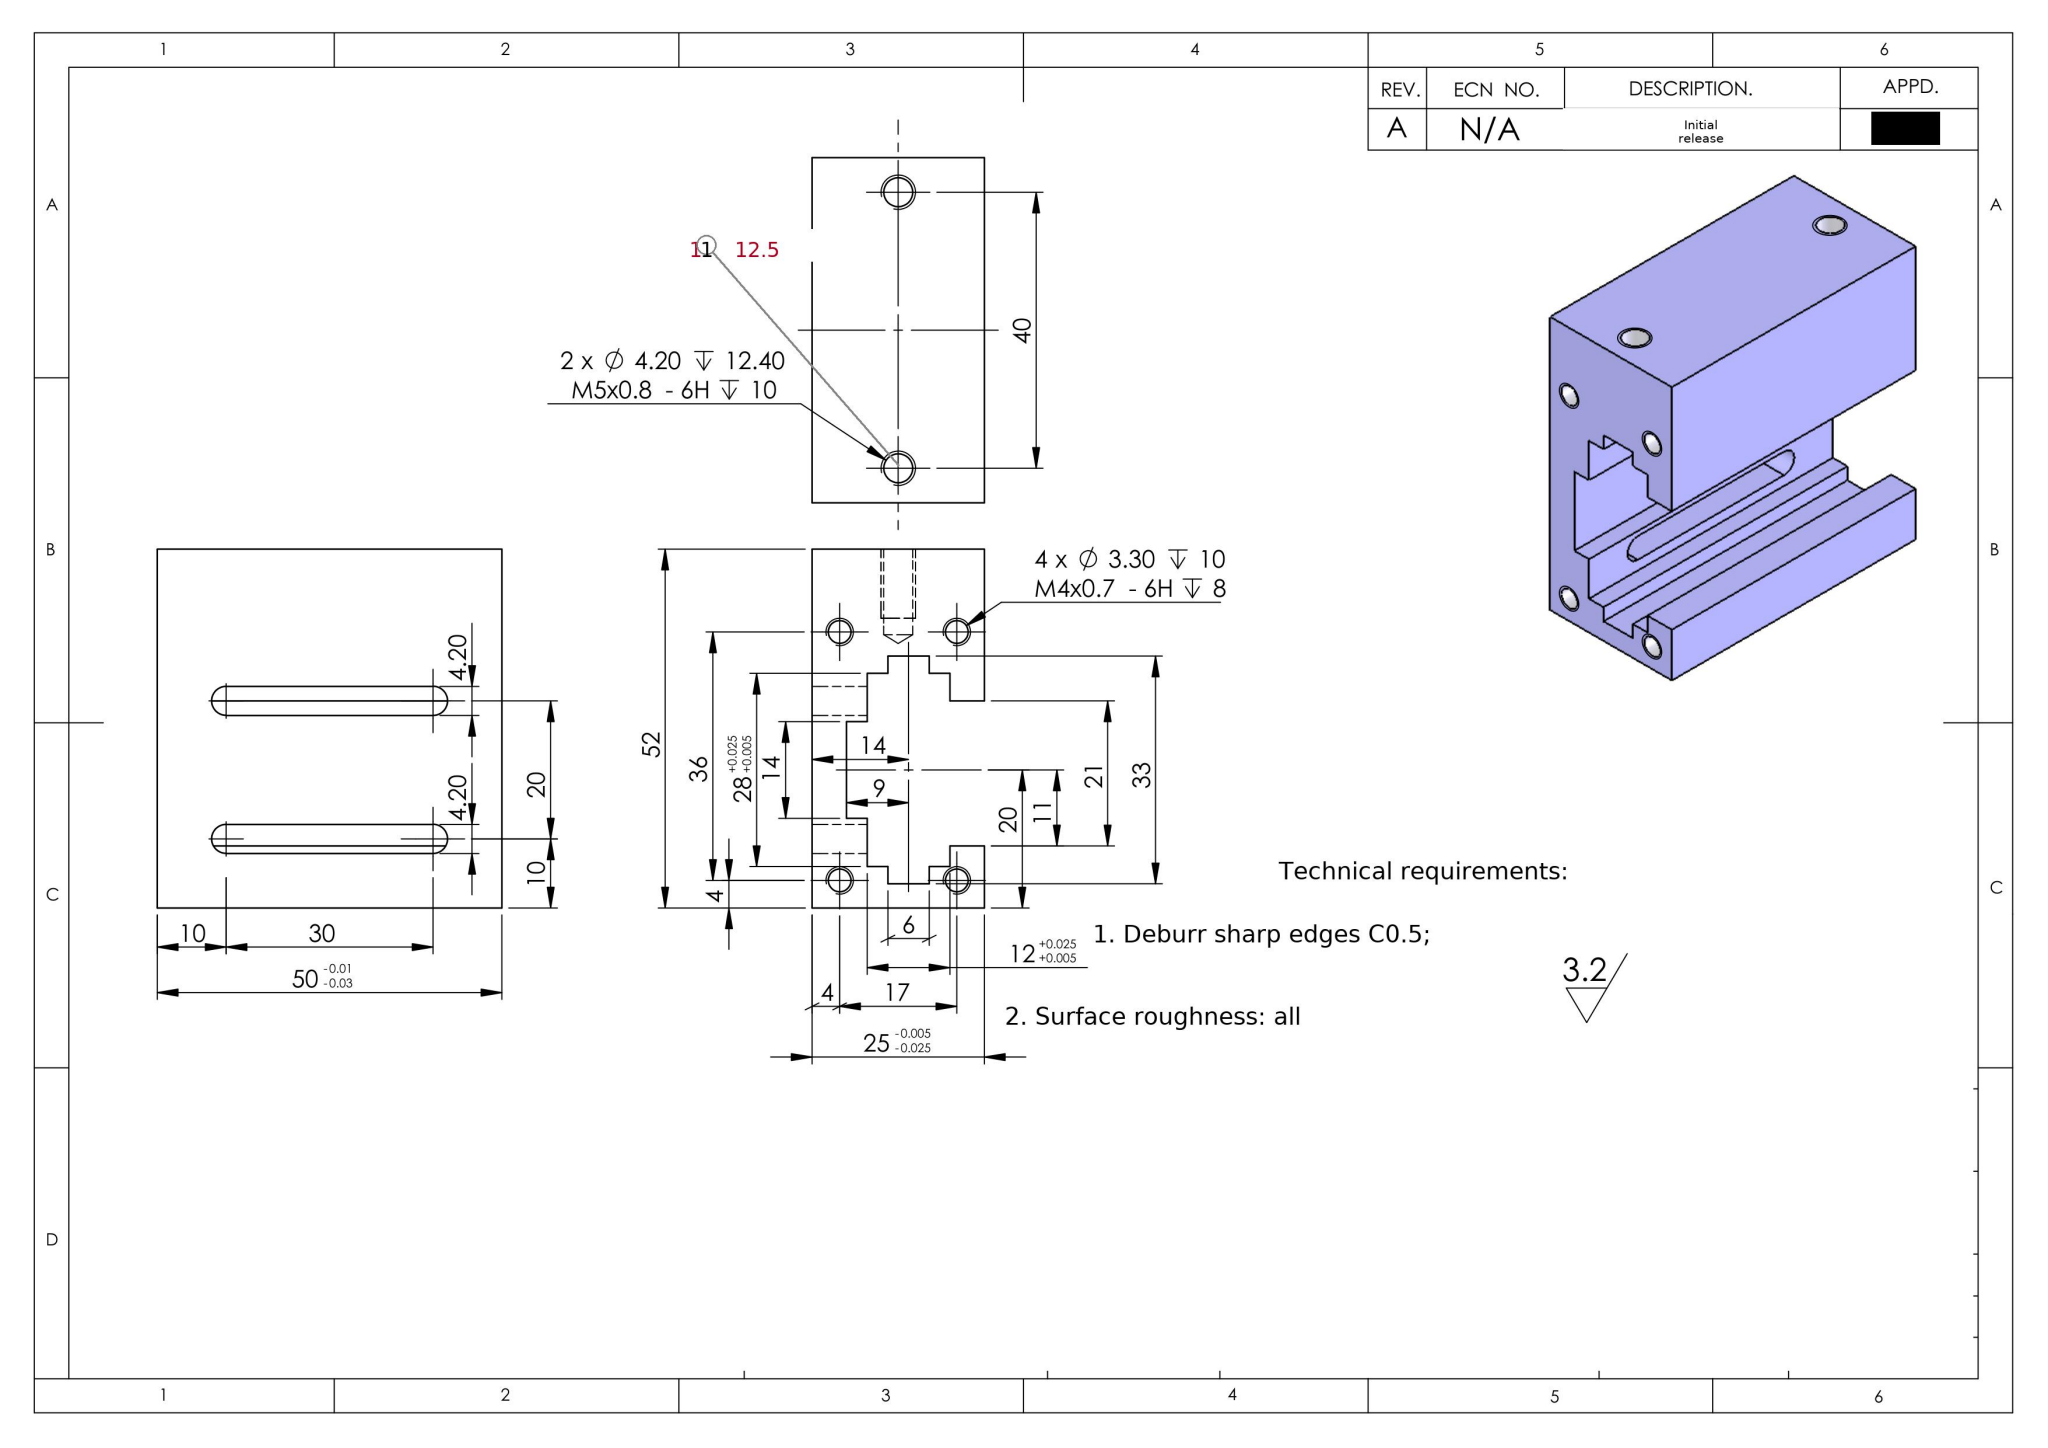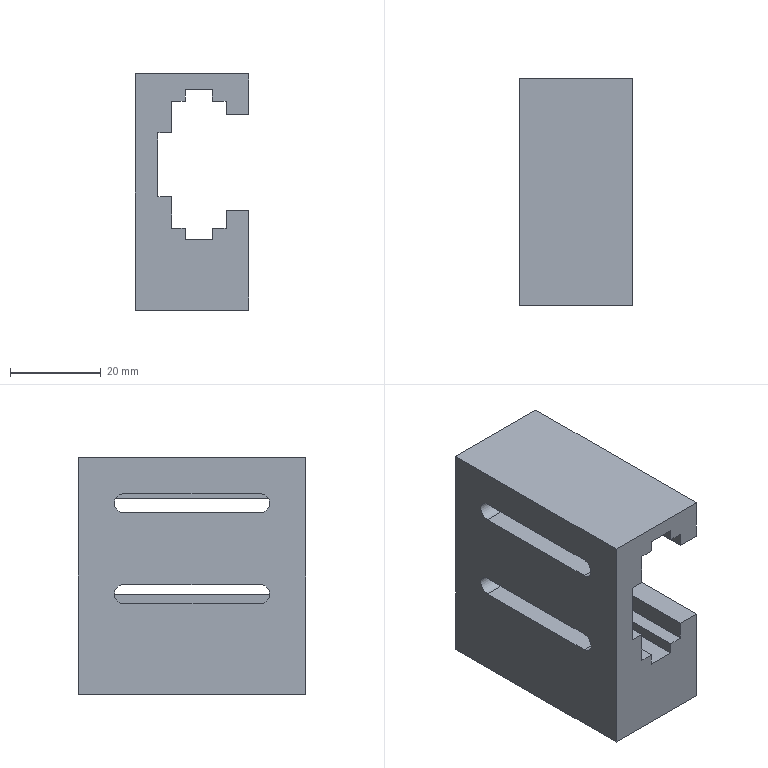Part | SolidWorks | mm | 1 solid | 58 faces | box 25 x 50 x 52 mm | volume 36404 mm3 | plane 30 | cylinder 16 | cone 12 | commonest cylinder face diameters 4.2 x8 3.3 x8
build123d program:
from build123d import *

# Parameters (mm, degrees)
EXTRUDE1_DEPTH        = 50
SKETCH3_W             = 3
SKETCH3_H             = 14
CUT_EXTRUDE2_DEPTH    = 75.115
CUT_EXTRUDE3_REACH    = 78.348
SKETCH6_W             = 6
SKETCH6_H             = 50
EXTRUDE2_DEPTH        = 3
SKETCH7_W             = 3
SKETCH7_H             = 10
EXTRUDE3_DEPTH        = 50
SKETCH8_W             = 5
SKETCH8_H             = 50
EXTRUDE4_DEPTH        = 14
EXTRUDE5_DEPTH        = 50
SKETCH10_W            = 3
SKETCH10_H            = 10
EXTRUDE6_DEPTH        = 50
SKETCH11_W            = 6
SKETCH11_H            = 2.5
CUT_EXTRUDE4_DEPTH    = 50
M4_TAPPED_HOLE1_D     = 3.3
M4_TAPPED_HOLE1_DEPTH = 10
M4_TAPPED_HOLE1_TIP   = 0.9914
EXTRUDE7_DEPTH        = 50
M5_TAPPED_HOLE1_D     = 4.2
M5_TAPPED_HOLE1_DEPTH = 12.4
M5_TAPPED_HOLE1_TIP   = 1.262


with BuildPart() as part:
    # Sketch1 → Extrude1 (new body)
    with BuildSketch(Plane(origin=(0, 0, 0), x_dir=(1, 0, 0), z_dir=(0, 1, 0))):
        Polygon((-8, 0), (-8, 52), (17, 52), (17, 44), (0, 44), (0, 0), align=None)
    extrude(amount=EXTRUDE1_DEPTH)

    # Sketch3 → Cut-Extrude2 (cut, through all)
    with BuildSketch(Plane.XZ):
        with Locations((-1.5, -20)):
            Rectangle(SKETCH3_W, SKETCH3_H)
    extrude(amount=-CUT_EXTRUDE2_DEPTH, mode=Mode.SUBTRACT)

    # Sketch5 → Cut-Extrude3 (cut, up to next)
    with BuildSketch(Plane.ZY.offset(8), mode=Mode.PRIVATE) as cut_extrude3_sk1:
        with BuildLine():
            Line((-32.1, 40), (-32.1, 10))
            ThreePointArc((-32.1, 10), (-30, 7.9), (-27.9, 10))
            Line((-27.9, 10), (-27.9, 40))
            ThreePointArc((-27.9, 40), (-30, 42.1), (-32.1, 40))
        make_face()
    cut_extrude3_tool1 = extrude(cut_extrude3_sk1.sketch, amount=-CUT_EXTRUDE3_REACH, mode=Mode.PRIVATE) & part.part
    # Sketch5 → Cut-Extrude3 (cut, up to next)
    with BuildSketch(Plane.ZY.offset(8), mode=Mode.PRIVATE) as cut_extrude3_sk2:
        with BuildLine():
            Line((-12.1, 40), (-12.1, 10))
            ThreePointArc((-12.1, 10), (-10, 7.9), (-7.9, 10))
            Line((-7.9, 10), (-7.9, 40))
            ThreePointArc((-7.9, 40), (-10, 42.1), (-12.1, 40))
        make_face()
    cut_extrude3_tool2 = extrude(cut_extrude3_sk2.sketch, amount=-CUT_EXTRUDE3_REACH, mode=Mode.PRIVATE) & part.part
    add(cut_extrude3_tool1.solids().sort_by_distance((-8, 25, -30))[0], mode=Mode.SUBTRACT)
    add(cut_extrude3_tool2.solids().sort_by_distance((-8, 25, -10))[0], mode=Mode.SUBTRACT)

    # Sketch6 → Extrude2 (add)
    with BuildSketch(Plane(origin=(0, 0, 0), x_dir=(0, 0, -1), z_dir=(1, 0, 0))):
        with Locations((3, 25)):
            Rectangle(SKETCH6_W, SKETCH6_H)
    extrude(amount=EXTRUDE2_DEPTH)

    # Sketch7 → Extrude3 (add)
    with BuildSketch(Plane(origin=(0, 50, 0), x_dir=(-1, 0, 0), z_dir=(0, 1, 0))):
        with Locations((-1.5, -39)):
            Rectangle(SKETCH7_W, SKETCH7_H)
    extrude(amount=-EXTRUDE3_DEPTH)

    # Sketch8 → Extrude4 (add)
    with BuildSketch(Plane.XY.offset(-44)):
        with Locations((14.5, 25)):
            Rectangle(SKETCH8_W, SKETCH8_H)
    extrude(amount=EXTRUDE4_DEPTH)

    # Sketch9 → Extrude5 (add)
    with BuildSketch(Plane.XZ):
        Polygon((17, 0), (17, -9), (12, -9), (12, -6), (3, -6), (3, 0), align=None)
    extrude(amount=-EXTRUDE5_DEPTH)

    # Sketch10 → Extrude6 (add)
    with BuildSketch(Plane.XZ):
        with Locations((10.5, -39)):
            Rectangle(SKETCH10_W, SKETCH10_H)
    extrude(amount=-EXTRUDE6_DEPTH)

    # Sketch11 → Cut-Extrude4 (cut)
    with BuildSketch(Plane.XZ):
        with Locations((6, -4.75)):
            Rectangle(SKETCH11_W, SKETCH11_H)
    extrude(amount=-CUT_EXTRUDE4_DEPTH, mode=Mode.SUBTRACT)

    # M4 Tapped Hole1
    with Locations(Plane(origin=(0, 50, 0), x_dir=(-1, 0, 0), z_dir=(0, 1, 0))):
        with Locations((4, -4), (-13, -4), (-13, -40), (4, -40)):
            Hole(M4_TAPPED_HOLE1_D / 2, depth=M4_TAPPED_HOLE1_DEPTH)
            with Locations((0, 0, -(M4_TAPPED_HOLE1_DEPTH + M4_TAPPED_HOLE1_TIP / 2))):  # 118° drill point
                Cone(0, M4_TAPPED_HOLE1_D / 2, M4_TAPPED_HOLE1_TIP, mode=Mode.SUBTRACT)

    # Sketch15 → Extrude7 (add)
    with BuildSketch(Plane.XZ):
        Polygon((9, -36.5), (3, -36.5), (3, -44), (9, -44), align=None)
    extrude(amount=-EXTRUDE7_DEPTH)

    # M5 Tapped Hole1
    with Locations(Plane(origin=(4.5, 45, -52), x_dir=(-1, 0, 0), z_dir=(0, 0, -1))):
        with Locations((0, 0), (0, -40)):
            Hole(M5_TAPPED_HOLE1_D / 2, depth=M5_TAPPED_HOLE1_DEPTH)
            with Locations((0, 0, -(M5_TAPPED_HOLE1_DEPTH + M5_TAPPED_HOLE1_TIP / 2))):  # 118° drill point
                Cone(0, M5_TAPPED_HOLE1_D / 2, M5_TAPPED_HOLE1_TIP, mode=Mode.SUBTRACT)


solid = part.part